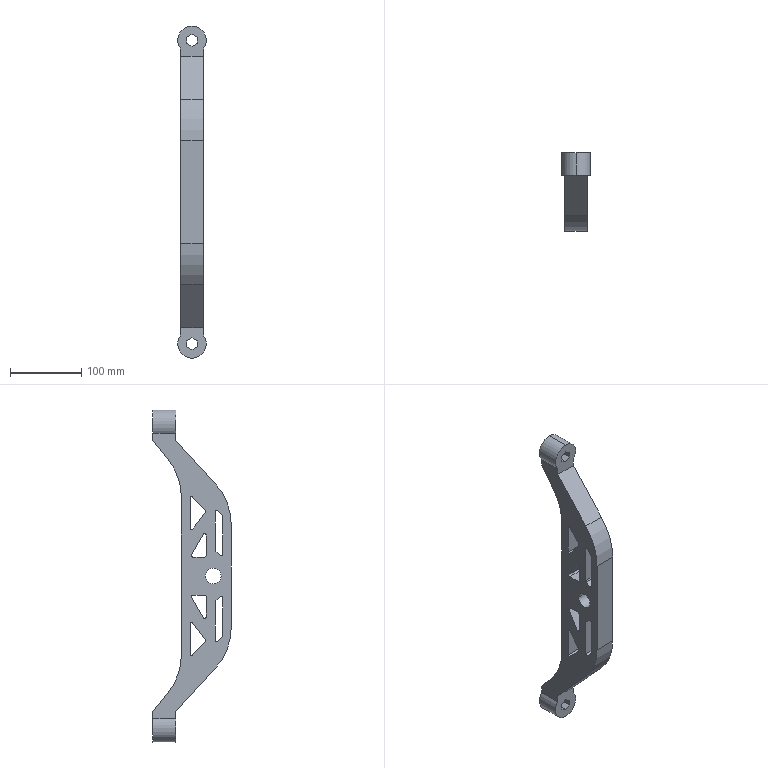Component | SolidWorks | FrontGuideWheel-1_GuideWheelBracket2-1 | 1 solid | 75 faces | box 40 x 110 x 465.28 mm | volume 645232 mm3 | plane 44 | cylinder 31 | commonest cylinder face diameters 4 x22 40 x3 22 x2 170 x2 167 x2
build123d program:
from build123d import *

# Parameters (mm, degrees)
SKETCH1_R           = 11
BOSS_EXTRUDE1_DEPTH = 31
SKETCH2_R           = 20
BOSS_EXTRUDE2_DEPTH = 32
FILLET1_R           = 2


with BuildPart() as part:
    # Sketch1 → Boss-Extrude1 (new body)
    with BuildSketch(Plane(origin=(0, 0, 0), x_dir=(1, 0, 0), z_dir=(0, 1, 0))):
        with BuildLine():
            Line((-71.841, 0), (71.841, 0))
            ThreePointArc((71.841, 0), (102.654, 5.782), (129.276, 22.34))
            Line((129.276, 22.34), (190, 78))
            Line((190, 78), (200, 78))
            Line((200, 78), (200, 110))
            Line((200, 110), (190, 110))
            Line((190, 110), (163.101, 88.397))
            ThreePointArc((163.101, 88.397), (138.529, 74.733), (110.815, 70))
            Line((110.815, 70), (-110.815, 70))
            ThreePointArc((-110.815, 70), (-138.529, 74.733), (-163.101, 88.397))
            Line((-163.101, 88.397), (-190, 110))
            Line((-190, 110), (-200, 110))
            Line((-200, 110), (-200, 78))
            Line((-200, 78), (-190, 78))
            Line((-190, 78), (-129.276, 22.34))
            ThreePointArc((-129.276, 22.34), (-102.654, 5.782), (-71.841, 0))
        make_face()
        with Locations(Location((0, 25.299, 0), (0, 0, 270))):
            Circle(SKETCH1_R, mode=Mode.SUBTRACT)
        Polygon((26.605, 57.56), (26.605, 35.324), (64.971, 35.324), align=None, mode=Mode.SUBTRACT)
        Polygon((61.047, 57.56), (90.694, 35.324), (114.238, 57.56), align=None, mode=Mode.SUBTRACT)
        Polygon((34.633, 22.34), (95.054, 22.34), (83.787, 11.636), (26.605, 11.636), align=None, mode=Mode.SUBTRACT)
        Polygon((-26.605, 11.636), (-34.633, 22.34), (-95.054, 22.34), (-83.787, 11.636), align=None, mode=Mode.SUBTRACT)
        Polygon((-114.238, 57.56), (-61.047, 57.56), (-90.694, 35.324), align=None, mode=Mode.SUBTRACT)
        Polygon((-64.971, 35.324), (-26.605, 57.56), (-26.605, 35.324), align=None, mode=Mode.SUBTRACT)
    extrude(amount=BOSS_EXTRUDE1_DEPTH)

    # Sketch2 → Boss-Extrude2 (add)
    with BuildSketch(Plane(origin=(0, 0, -110), x_dir=(-1, 0, 0), z_dir=(0, 0, -1))):
        with Locations((-212.639, 15.5)):
            Circle(SKETCH2_R)
        Polygon((-204.319, 15.5), (-208.479, 22.705), (-216.799, 22.705), (-220.959, 15.5), (-216.799, 8.295), (-208.479, 8.295), align=None, mode=Mode.SUBTRACT)
    boss_extrude2 = extrude(amount=-BOSS_EXTRUDE2_DEPTH)

    # Mirror1: Boss-Extrude2 across plane
    add(boss_extrude2.mirror(Plane(origin=(0, 0, 0), x_dir=(0, 0, 1), z_dir=(1, 0, 0))))

    # Fillet1
    fillet1_edges = [part.edges().sort_by_distance(p)[0] for p in [
        (-64.971, 15.5, -35.324),
        (-26.605, 15.5, -35.324),
        (-26.605, 15.5, -57.56),
        (64.971, 15.5, -35.324),
        (26.605, 15.5, -57.56),
        (26.605, 15.5, -35.324),
        (114.238, 15.5, -57.56),
        (61.047, 15.5, -57.56),
        (90.694, 15.5, -35.324),
        (83.787, 15.5, -11.636),
        (95.054, 15.5, -22.34),
        (34.633, 15.5, -22.34),
        (26.605, 15.5, -11.636),
        (-83.787, 15.5, -11.636),
        (-26.605, 15.5, -11.636),
        (-34.633, 15.5, -22.34),
        (-95.054, 15.5, -22.34),
        (-114.238, 15.5, -57.56),
        (-90.694, 15.5, -35.324),
        (-61.047, 15.5, -57.56),
    ]]
    fillet(fillet1_edges, radius=FILLET1_R)


solid = part.part

# Placed as in the assembly
solid = solid.moved(Location((544.259, 2.387, -216.572), (90, 0, 90)))